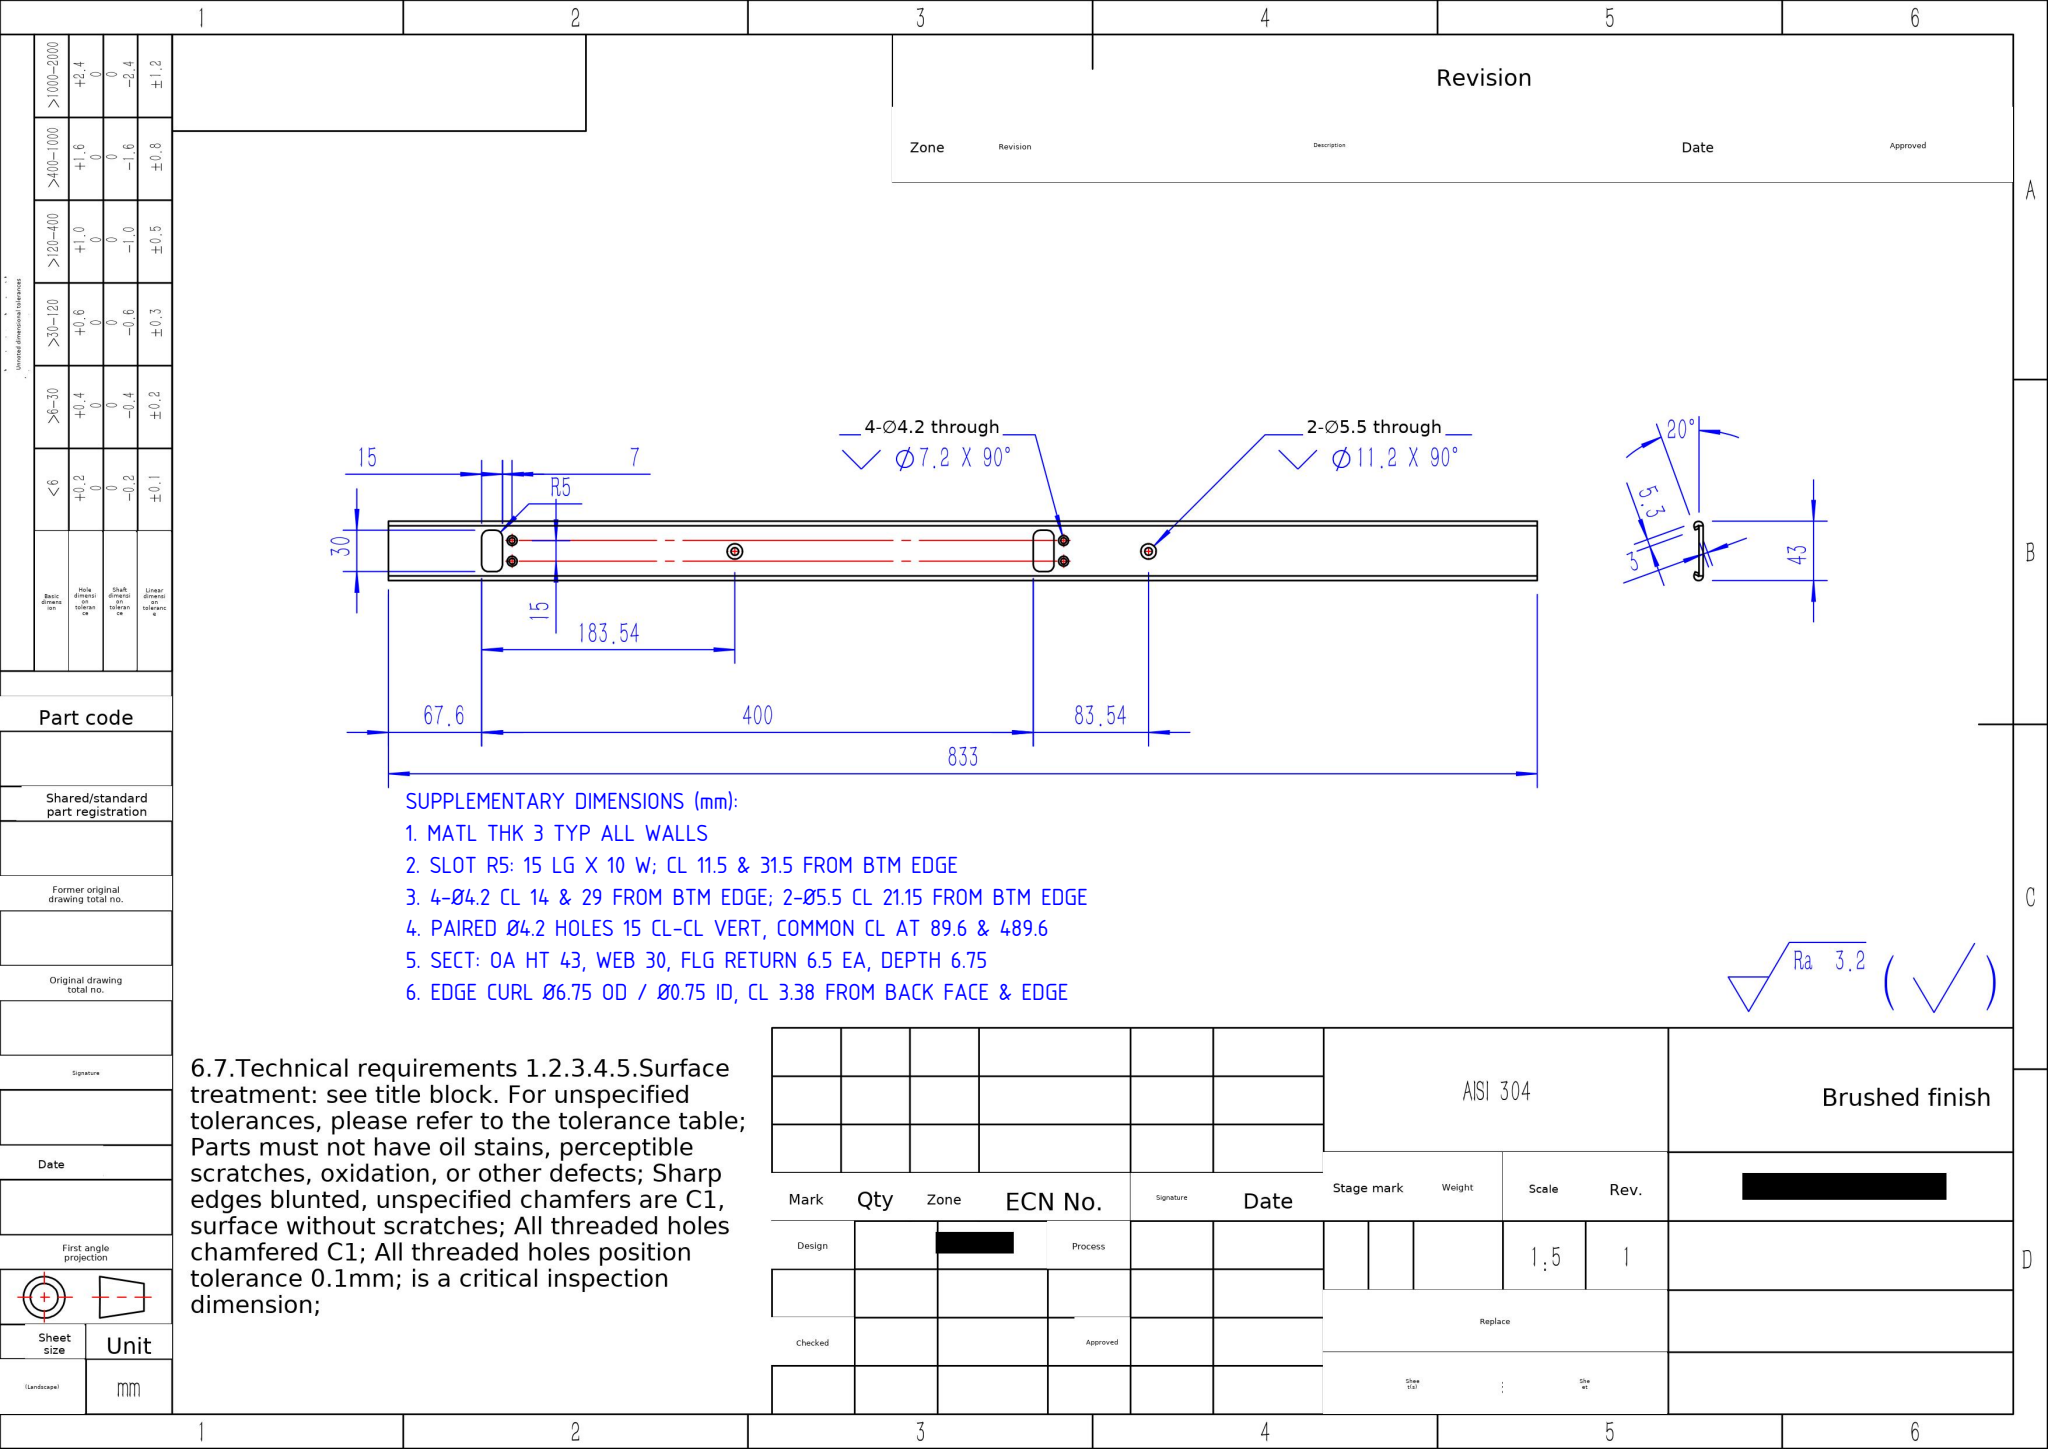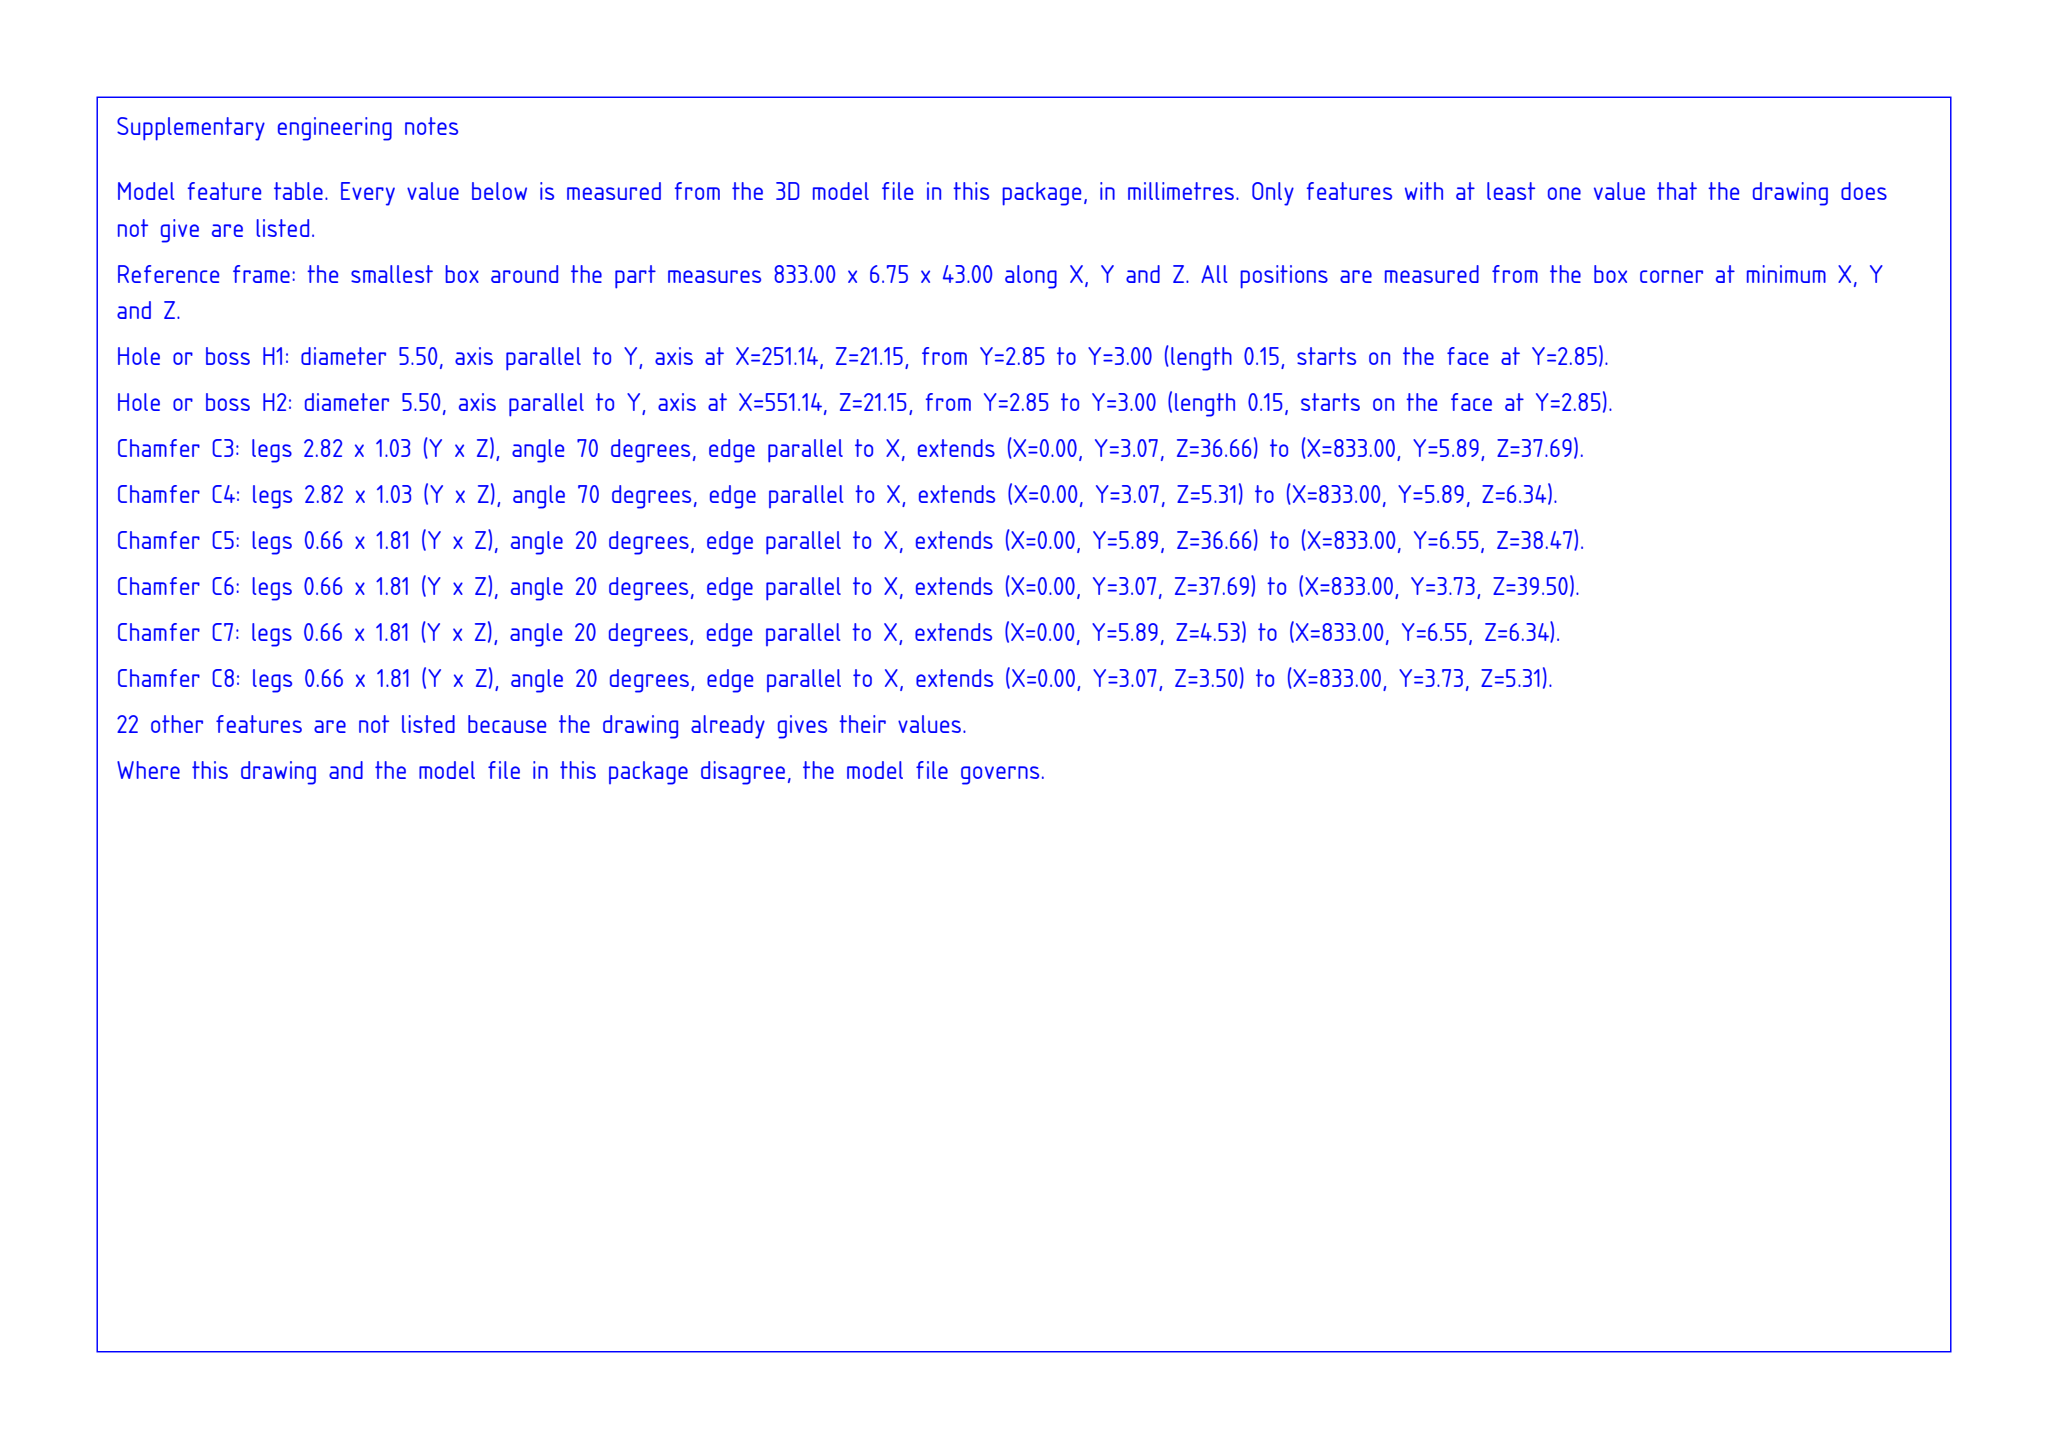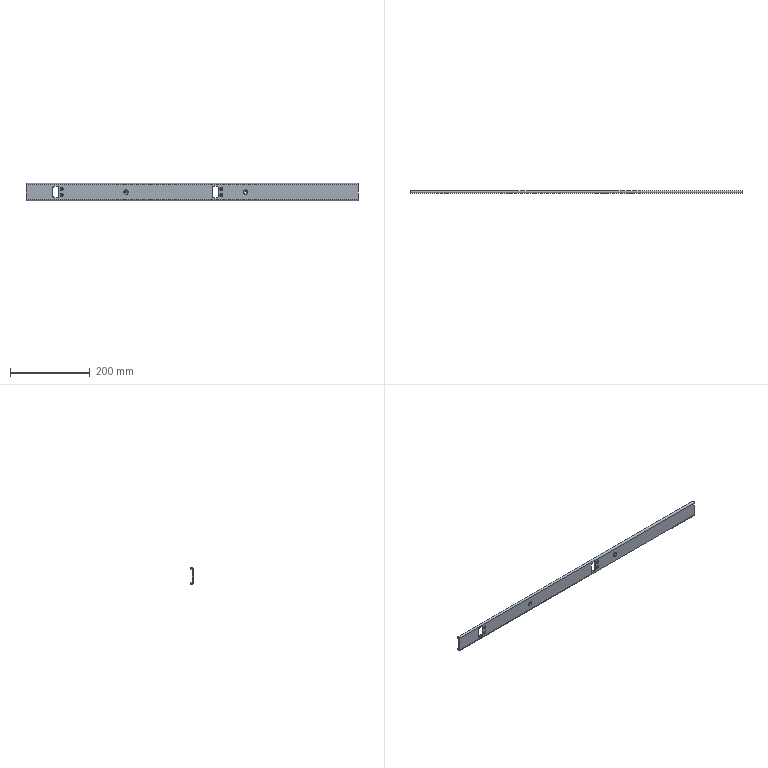Part | SolidWorks | mm | 1 solid | 62 faces | box 833 x 6.75 x 43 mm | volume 129788 mm3 | plane 26 | cylinder 24 | cone 12 | commonest cylinder face diameters 4.2 x8 10 x8 5.5 x4 6.75 x2 0.75 x2